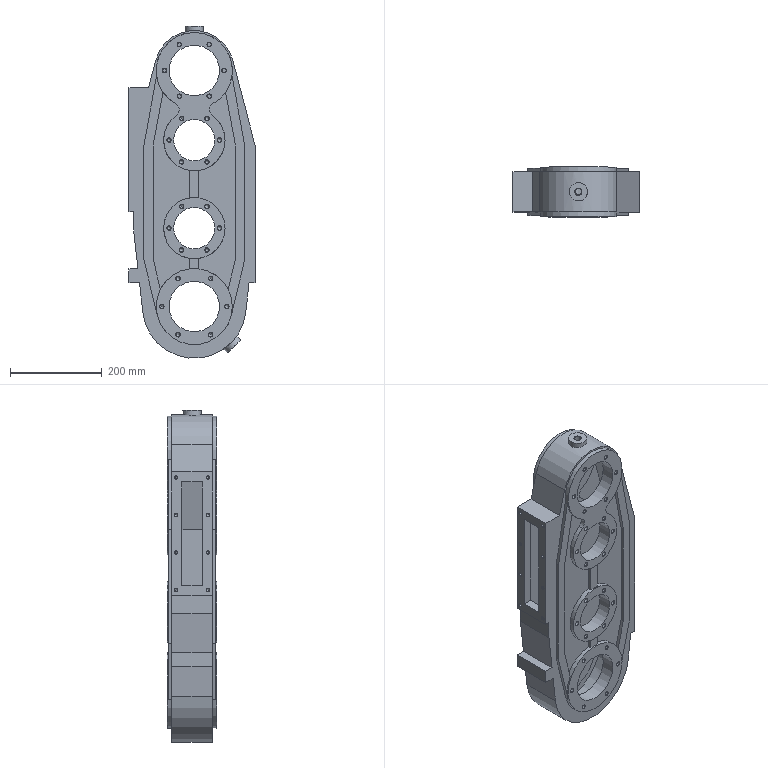Component | NX | SIDE_HOUSING | 1 solid | 308 faces | volume 5560283 mm3 | plane 112 | cylinder 98 | cone 96 | spline 2 | commonest cylinder face diameters 8.5 x48 166 x10 30.14 x8 134 x8 6.8 x8 90 x4 110 x4 40 x2